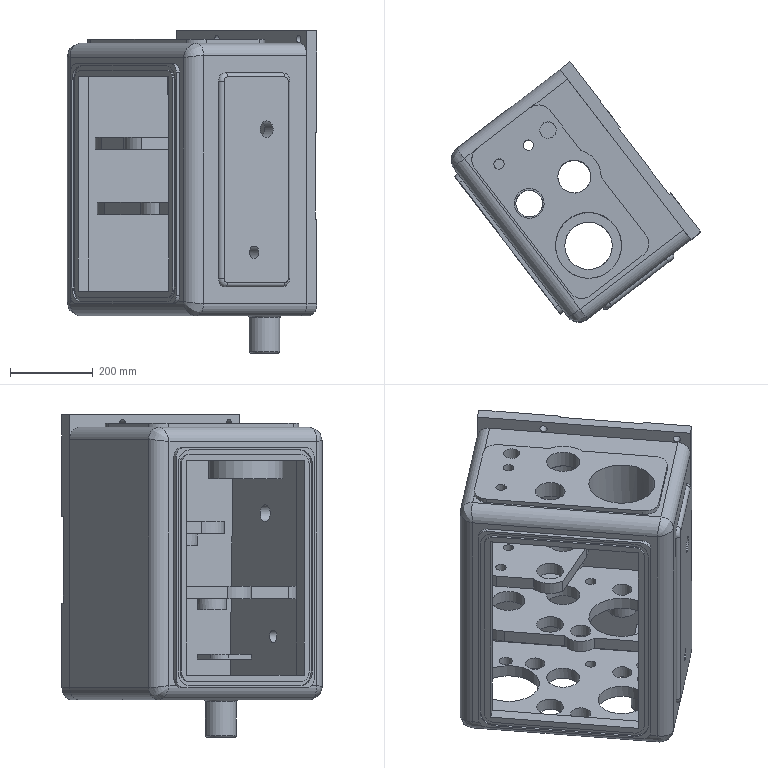Component | NX | ZHUZHOUXIANG2 | 6 solids | 202 faces | volume 37120152 mm3 | cylinder 94 | plane 91 | torus 8 | spline 6 | sphere 3 | commonest cylinder face diameters 70 x13 20 x12 80 x8 40 x7 60 x6 25 x6 47 x5 50 x4